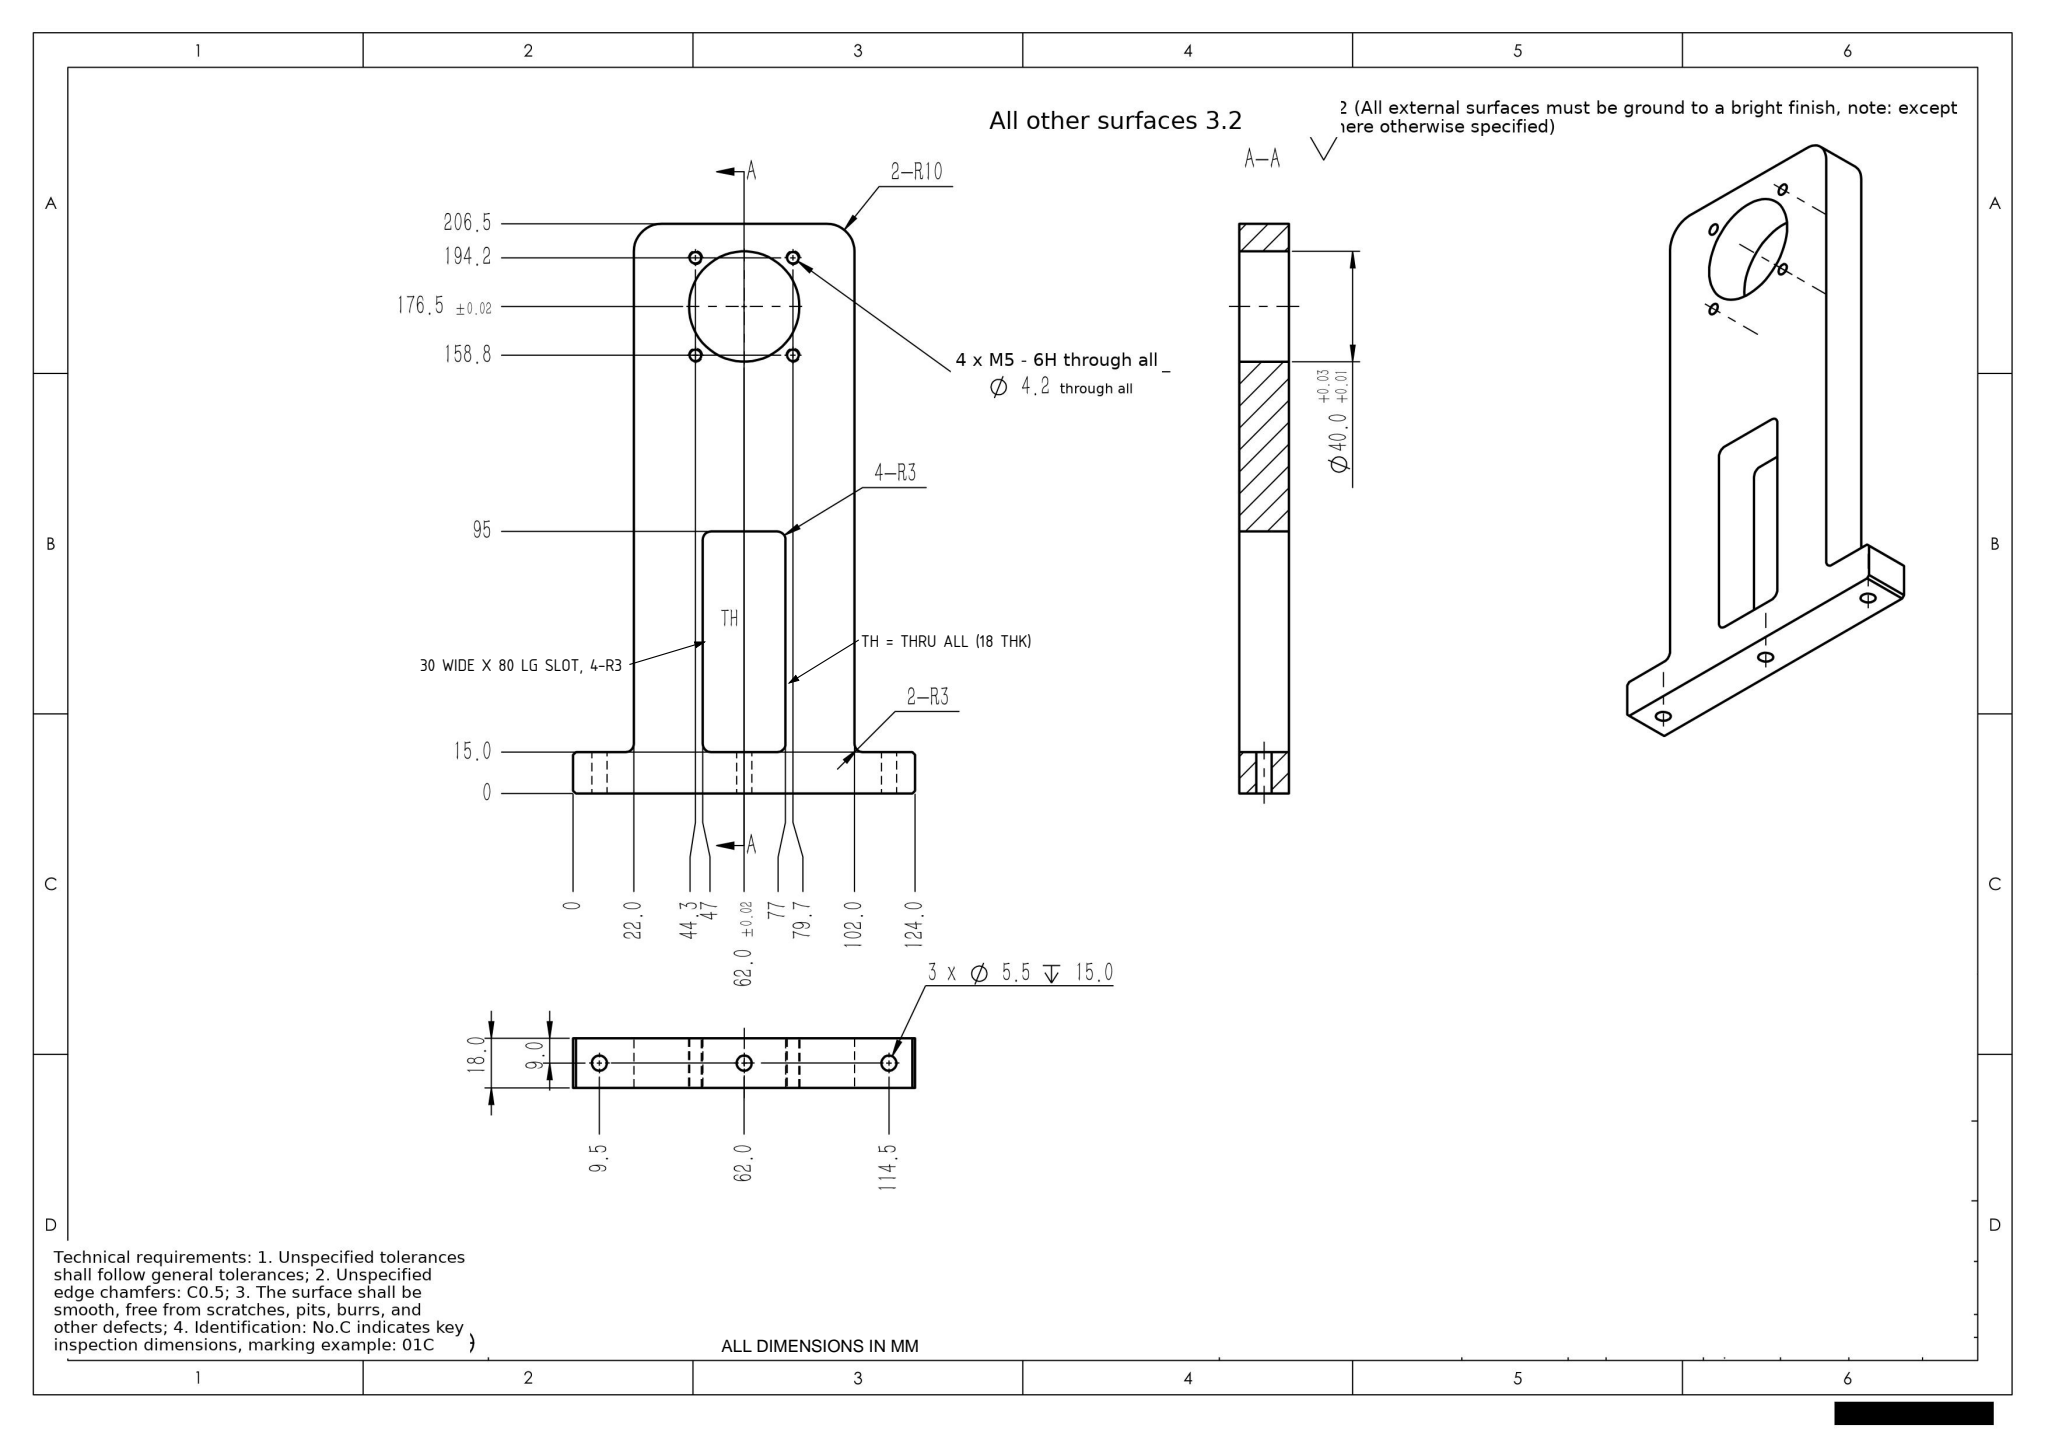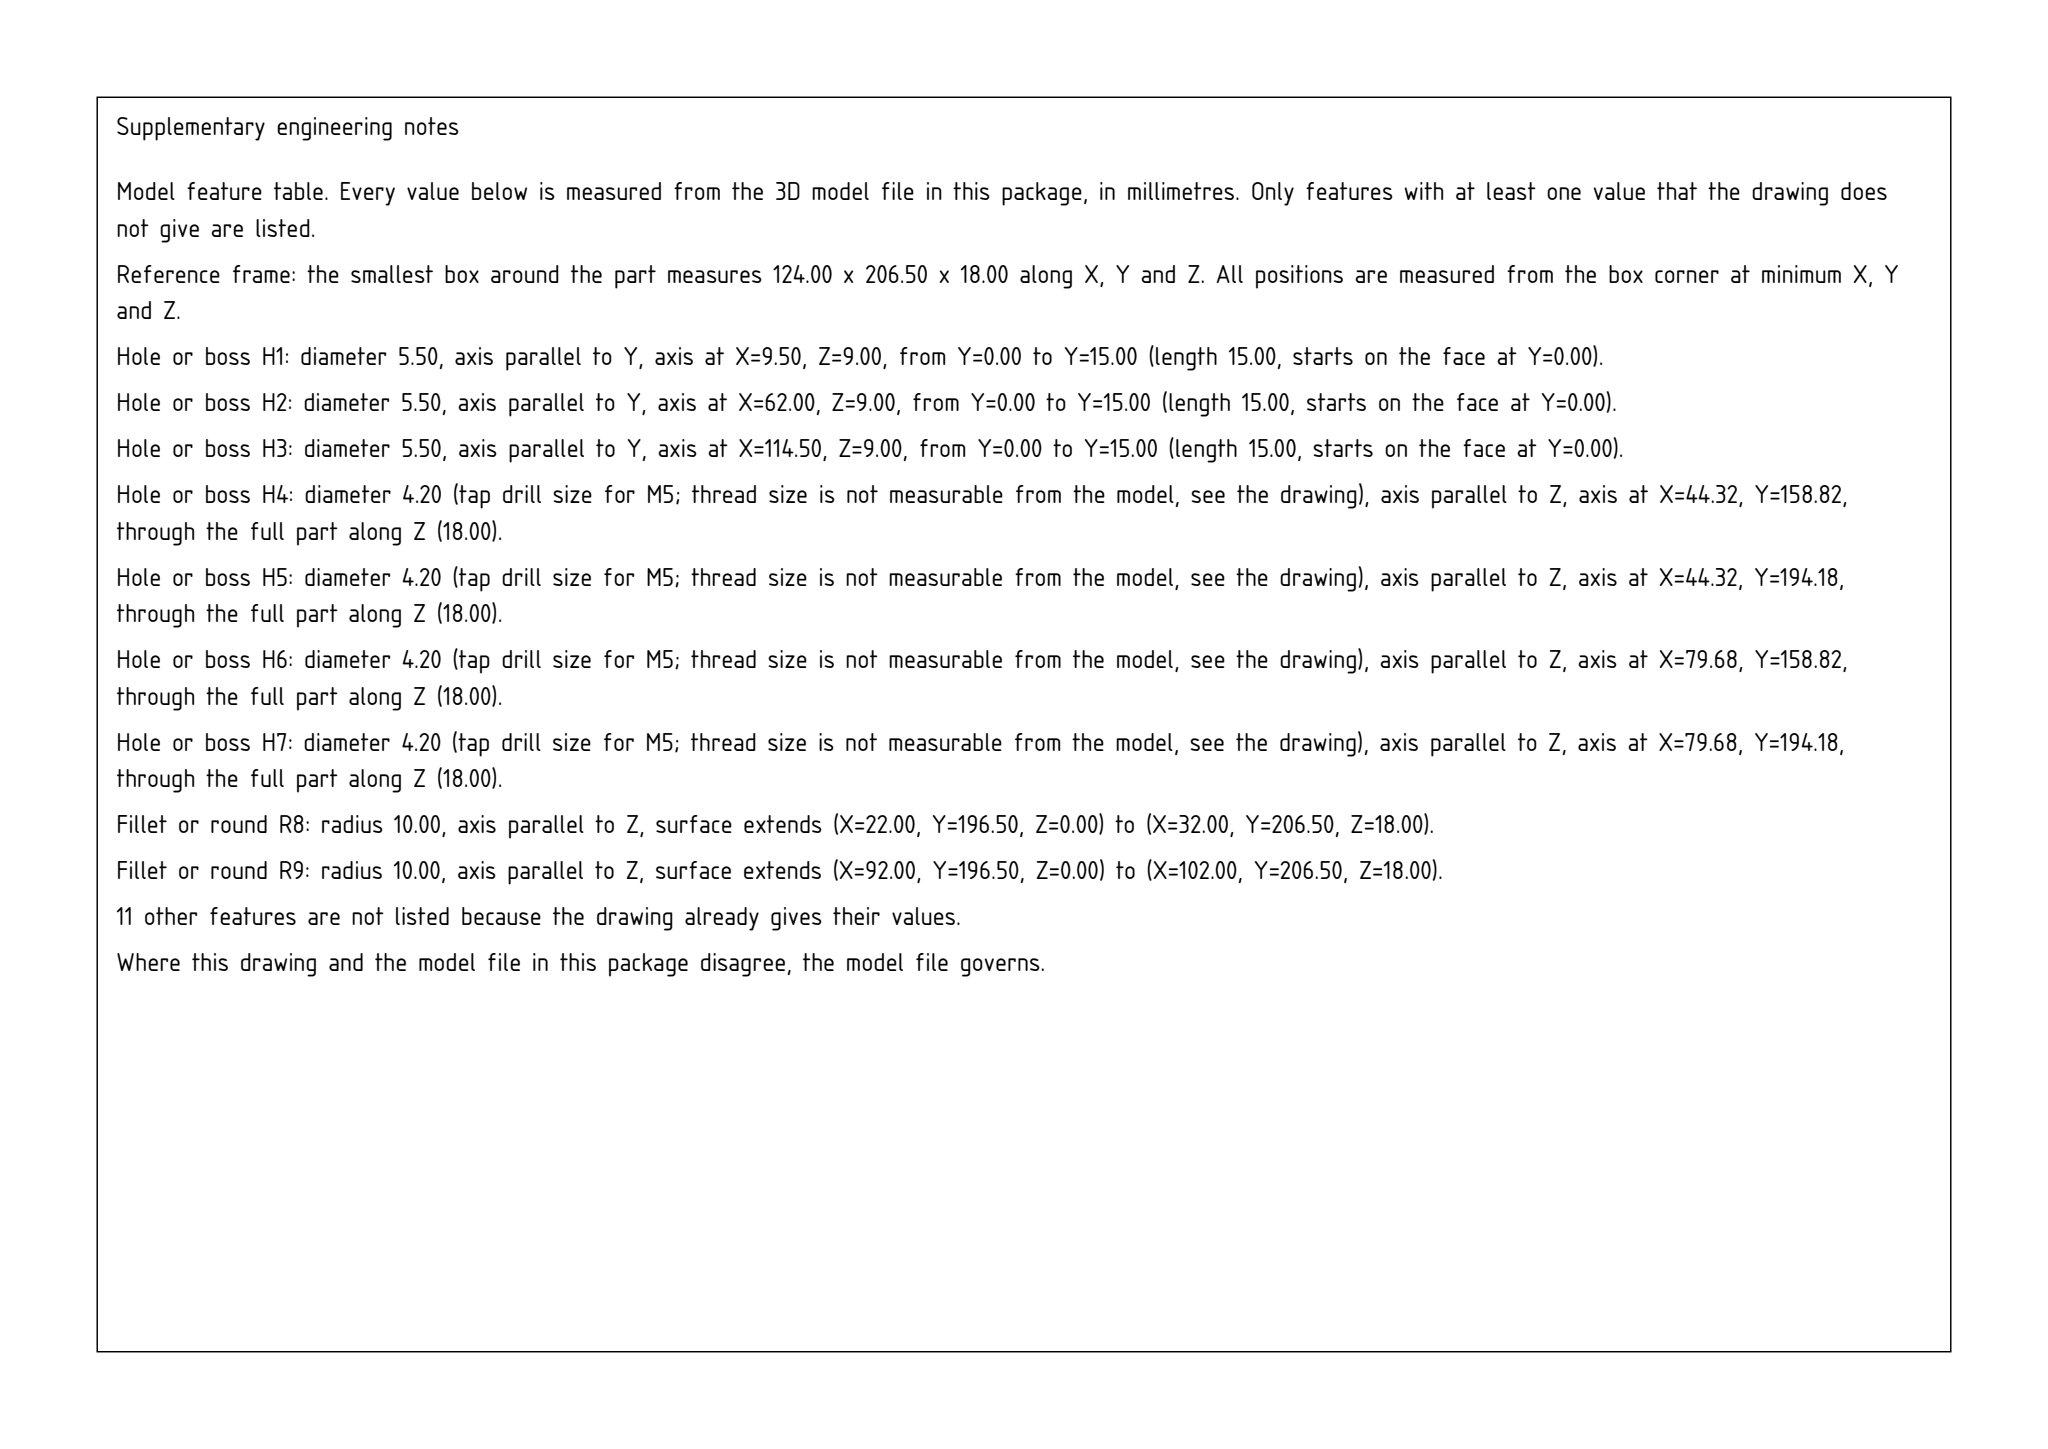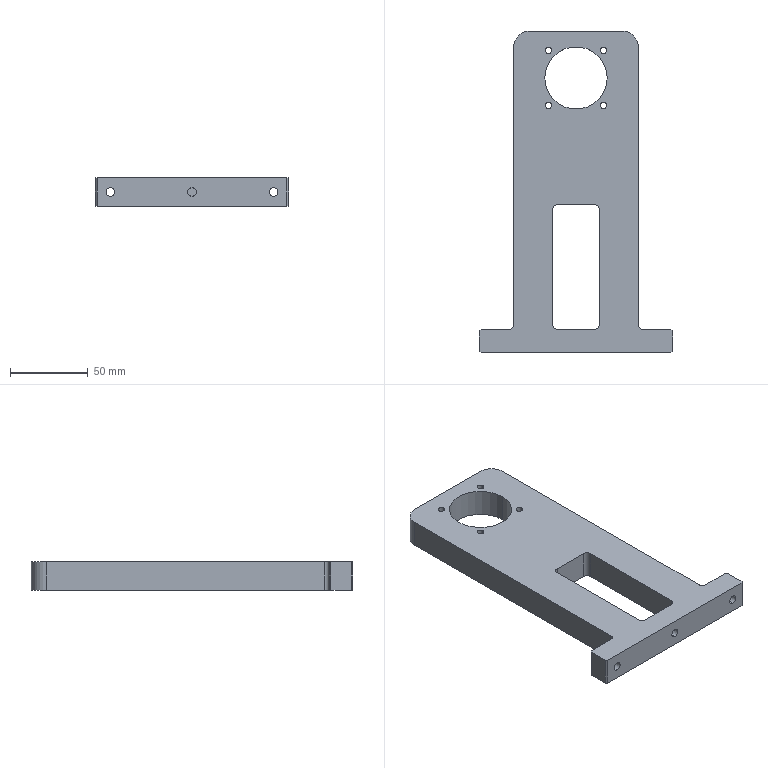Part | SolidWorks | mm | 1 solid | 42 faces | box 124 x 206.5 x 18 mm | volume 240754 mm3 | cylinder 24 | plane 18 | commonest cylinder face diameters 4.2 x8 5.5 x6 6 x6 40 x2 20 x2
Drawing notes:
TH SLOT: 30 WIDE (47 TO 77) x 80 LG, 15 TO 95, 4-R3 | from the solid: axis_planes x=47/77, y=15/95; slot walls bound TH feature
TH = THRU ALL (18 THK) | from the solid: bbox z=18; axis_planes z=0.0 and z=18.0, slot open both faces
build123d program:
from build123d import *

# Parameters (mm, degrees)
SKETCH1_W                      = 80
SKETCH1_H                      = 191.5
BOSS_EXTRUDE1_DEPTH            = 18
SKETCH2_W                      = 124
SKETCH2_H                      = 15
BOSS_EXTRUDE2_DEPTH            = 18
SKETCH3_R                      = 20
CUT_EXTRUDE2_DEPTH             = 129.193
CHAMFER1_SIZE                  = 1
FILLET1_R                      = 10
SKETCH7_W                      = 30
SKETCH7_H                      = 80
CUT_EXTRUDE4_DEPTH             = 129.193
F_5_5_5_5_DIAMETER_SLOT3_D     = 5.5
F_5_5_5_5_DIAMETER_SLOT3_DEPTH = 15
F_5_5_5_5_DIAMETER_SLOT3_TIP   = 1.652
FILLET2_R                      = 3
M5_TAPPED_HOLE2_D              = 4.2


with BuildPart() as part:
    # Sketch1 → Boss-Extrude1 (new body)
    with BuildSketch(Plane.XY):
        Rectangle(SKETCH1_W, SKETCH1_H)
    extrude(amount=BOSS_EXTRUDE1_DEPTH)

    # Sketch2 → Boss-Extrude2 (add)
    with BuildSketch(Plane.XY.offset(18)):
        with Locations((0, -103.25)):
            Rectangle(SKETCH2_W, SKETCH2_H)
    extrude(amount=-BOSS_EXTRUDE2_DEPTH)

    # Sketch3 → Cut-Extrude2 (cut, through all)
    with BuildSketch(Plane.XY.offset(18)):
        with Locations((0, 65.75)):
            Circle(SKETCH3_R)
    extrude(amount=-CUT_EXTRUDE2_DEPTH, mode=Mode.SUBTRACT)

    # Chamfer1
    chamfer1_edges = [part.edges().sort_by_distance(p)[0] for p in [
        (62, -110.75, 9),
        (62, -95.75, 9),
        (-62, -110.75, 9),
        (-62, -95.75, 9),
    ]]
    chamfer(chamfer1_edges, length=CHAMFER1_SIZE)

    # Fillet1
    fillet1_edges = [part.edges().sort_by_distance(p)[0] for p in [
        (40, 95.75, 9),
        (-40, 95.75, 9),
    ]]
    fillet(fillet1_edges, radius=FILLET1_R)

    # Sketch7 → Cut-Extrude4 (cut, through all)
    with BuildSketch(Plane.XY.offset(18)):
        with Locations((0, -55.75)):
            Rectangle(SKETCH7_W, SKETCH7_H)
    extrude(amount=-CUT_EXTRUDE4_DEPTH, mode=Mode.SUBTRACT)

    # 5.5 _5.5_ Diameter Slot3
    with Locations(Plane(origin=(0, -95.75, 0), x_dir=(1, 0, 0), z_dir=(0, 1, 0))):
        with Locations((-52.5, -9), (52.5, -9), (0, -9)):
            Hole(F_5_5_5_5_DIAMETER_SLOT3_D / 2, depth=F_5_5_5_5_DIAMETER_SLOT3_DEPTH)
            with Locations((0, 0, -(F_5_5_5_5_DIAMETER_SLOT3_DEPTH + F_5_5_5_5_DIAMETER_SLOT3_TIP / 2))):  # 118° drill point
                Cone(0, F_5_5_5_5_DIAMETER_SLOT3_D / 2, F_5_5_5_5_DIAMETER_SLOT3_TIP, mode=Mode.SUBTRACT)

    # Fillet2
    fillet2_edges = [part.edges().sort_by_distance(p)[0] for p in [
        (-15, -95.75, 9),
        (15, -95.75, 9),
        (15, -15.75, 9),
        (-15, -15.75, 9),
        (-40, -95.75, 9),
        (40, -95.75, 9),
    ]]
    fillet(fillet2_edges, radius=FILLET2_R)

    # M5 Tapped Hole2 (through all)
    with Locations(Plane(origin=(0, 0, 0), x_dir=(-1, 0, 0), z_dir=(0, 0, -1))):
        with Locations((17.678, 83.428), (17.678, 48.072), (-17.678, 48.072), (-17.678, 83.428)):
            Hole(M5_TAPPED_HOLE2_D / 2)


solid = part.part